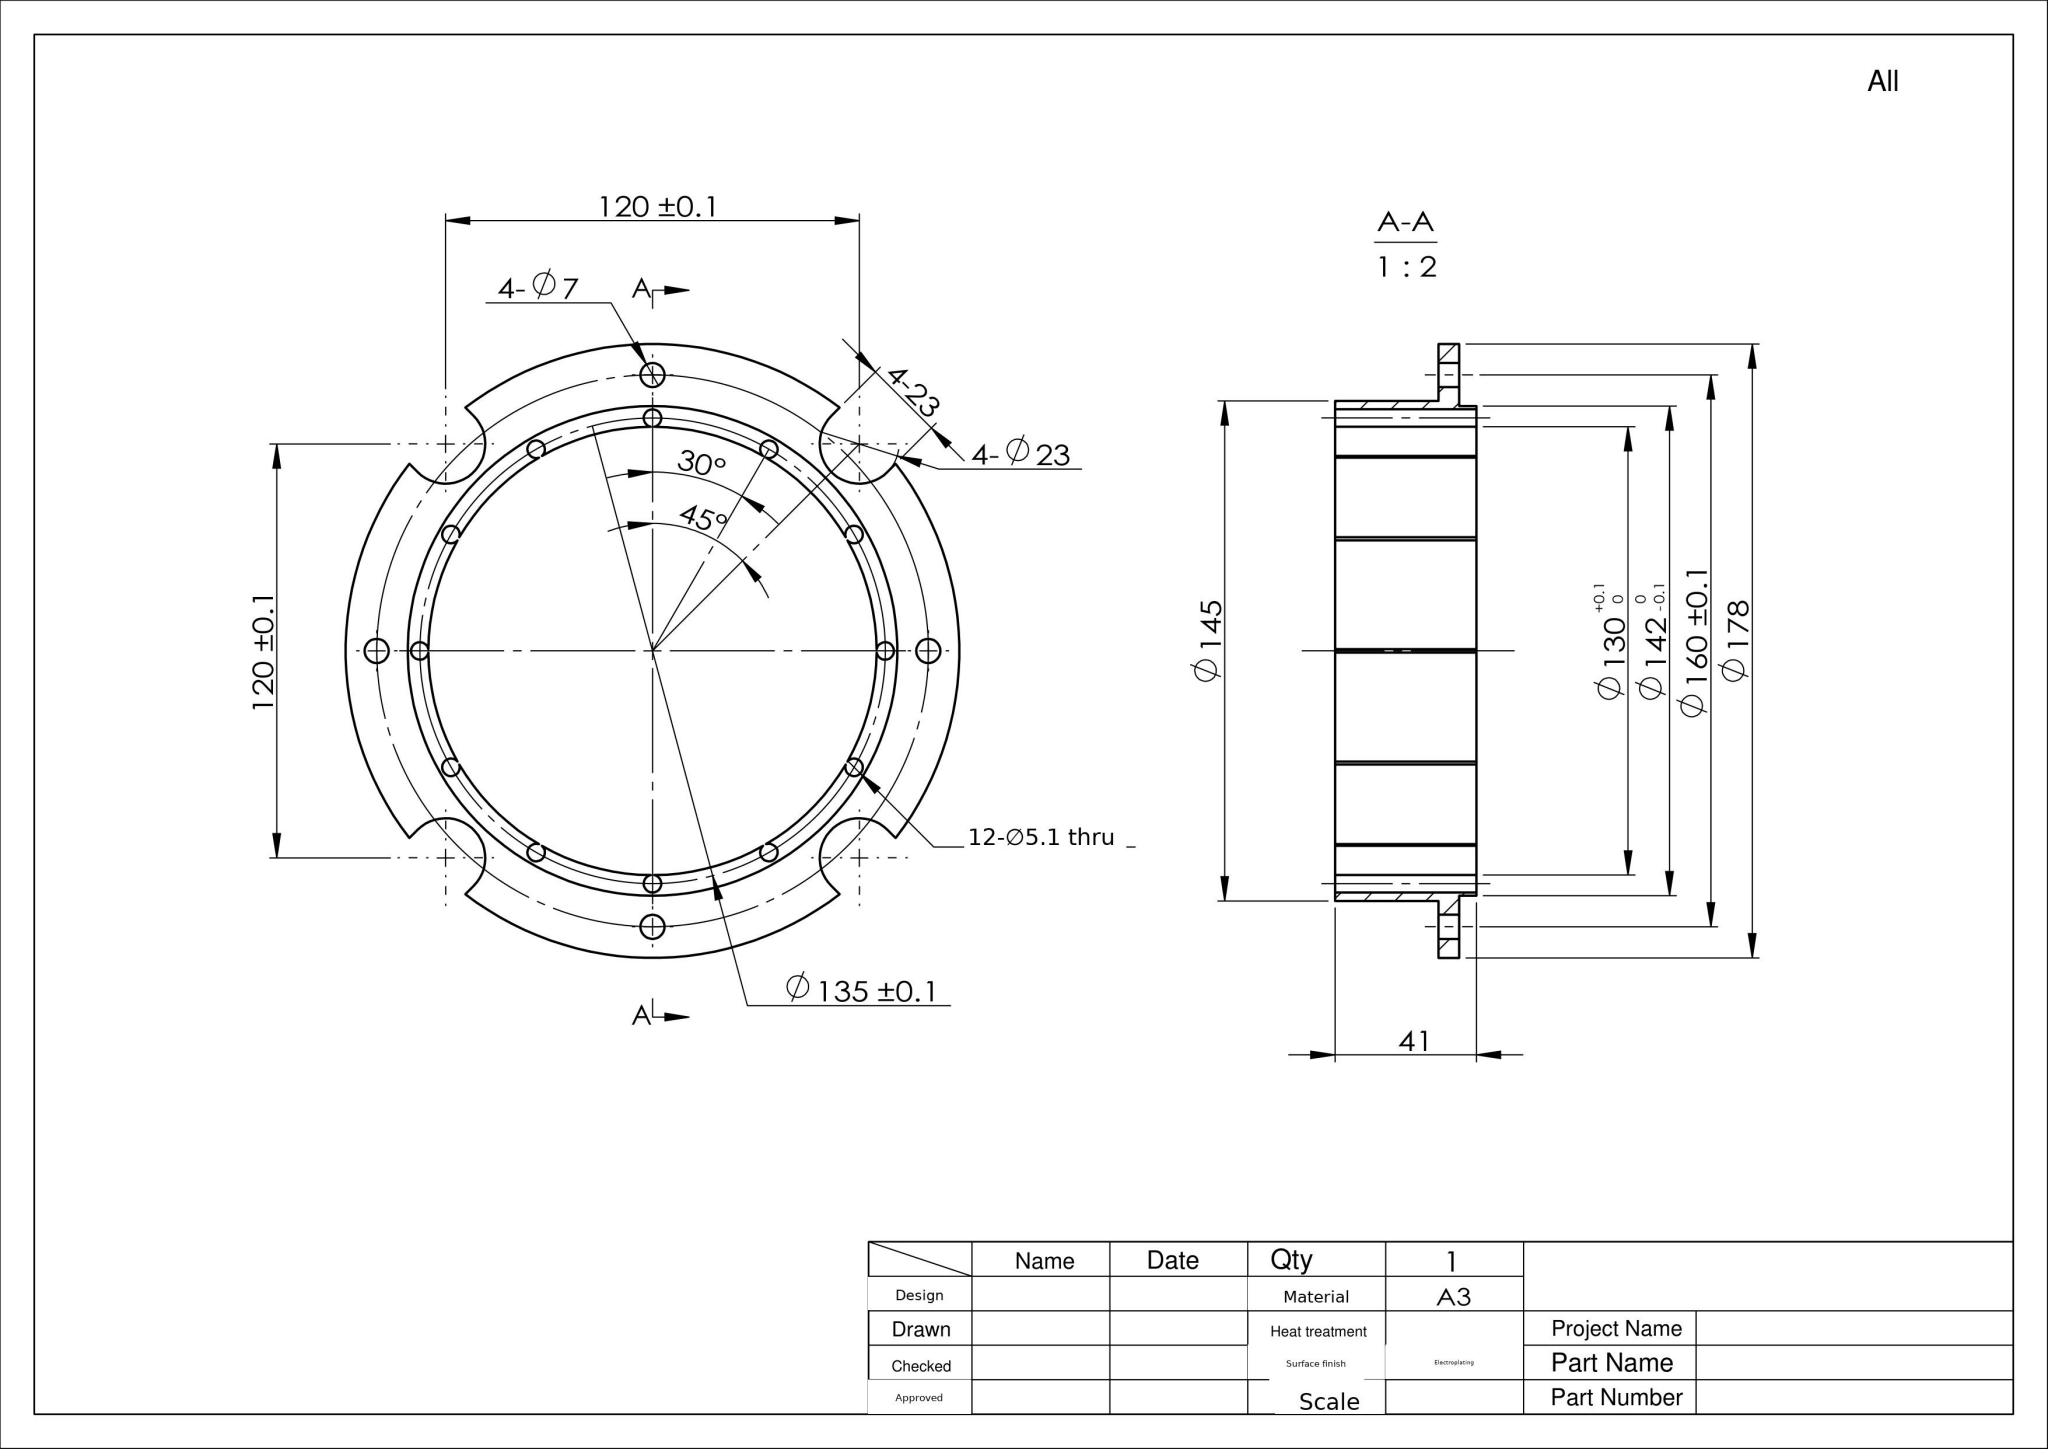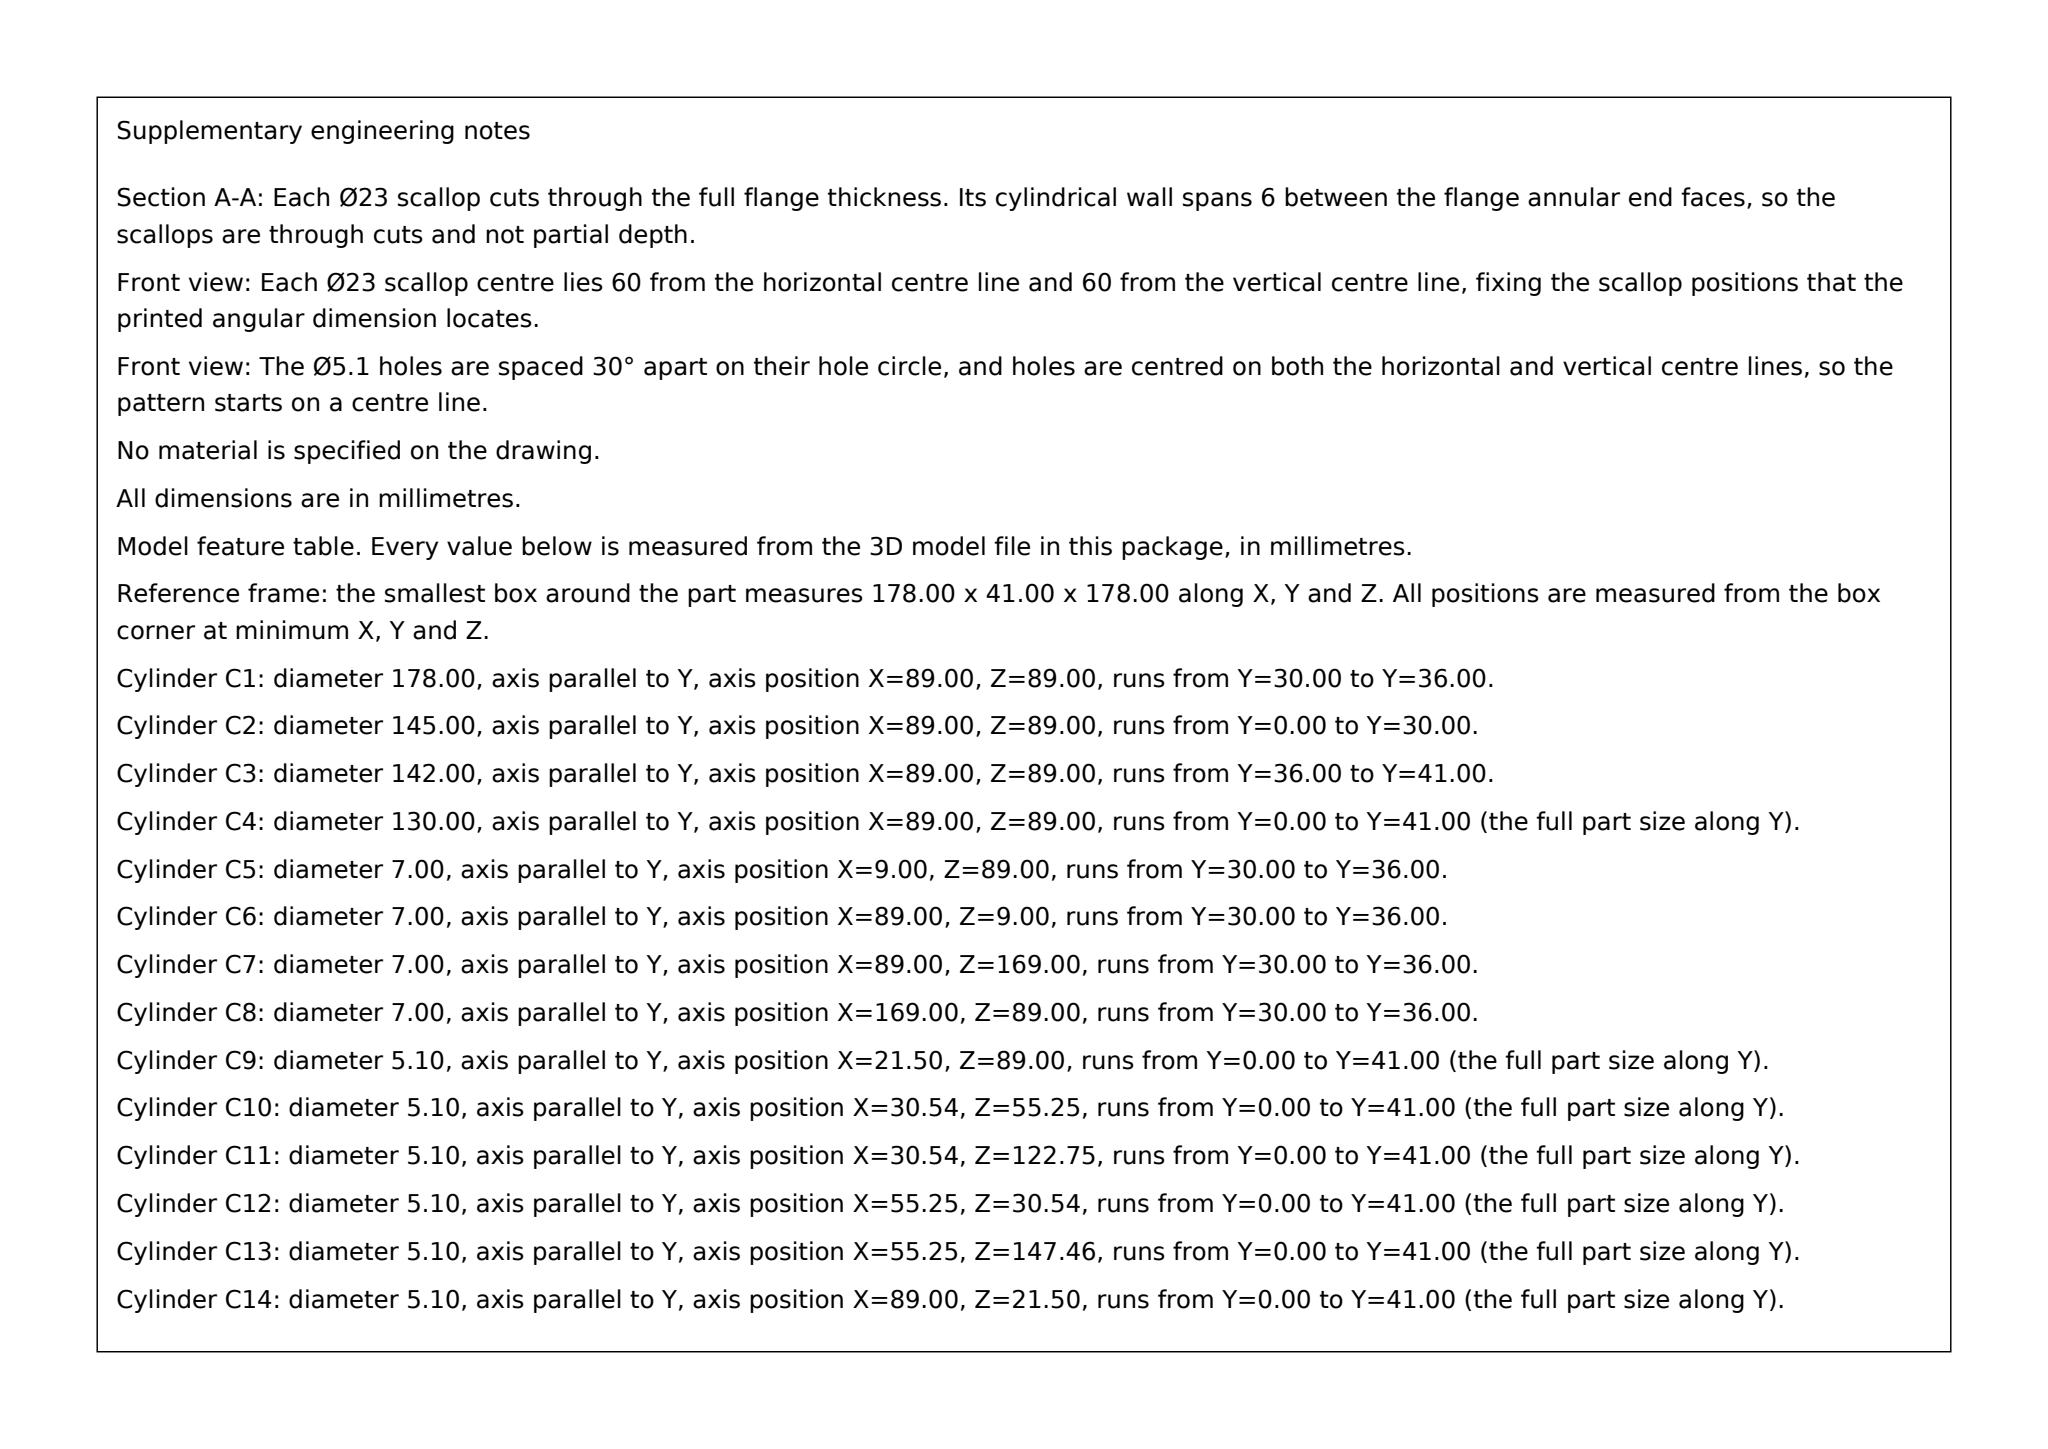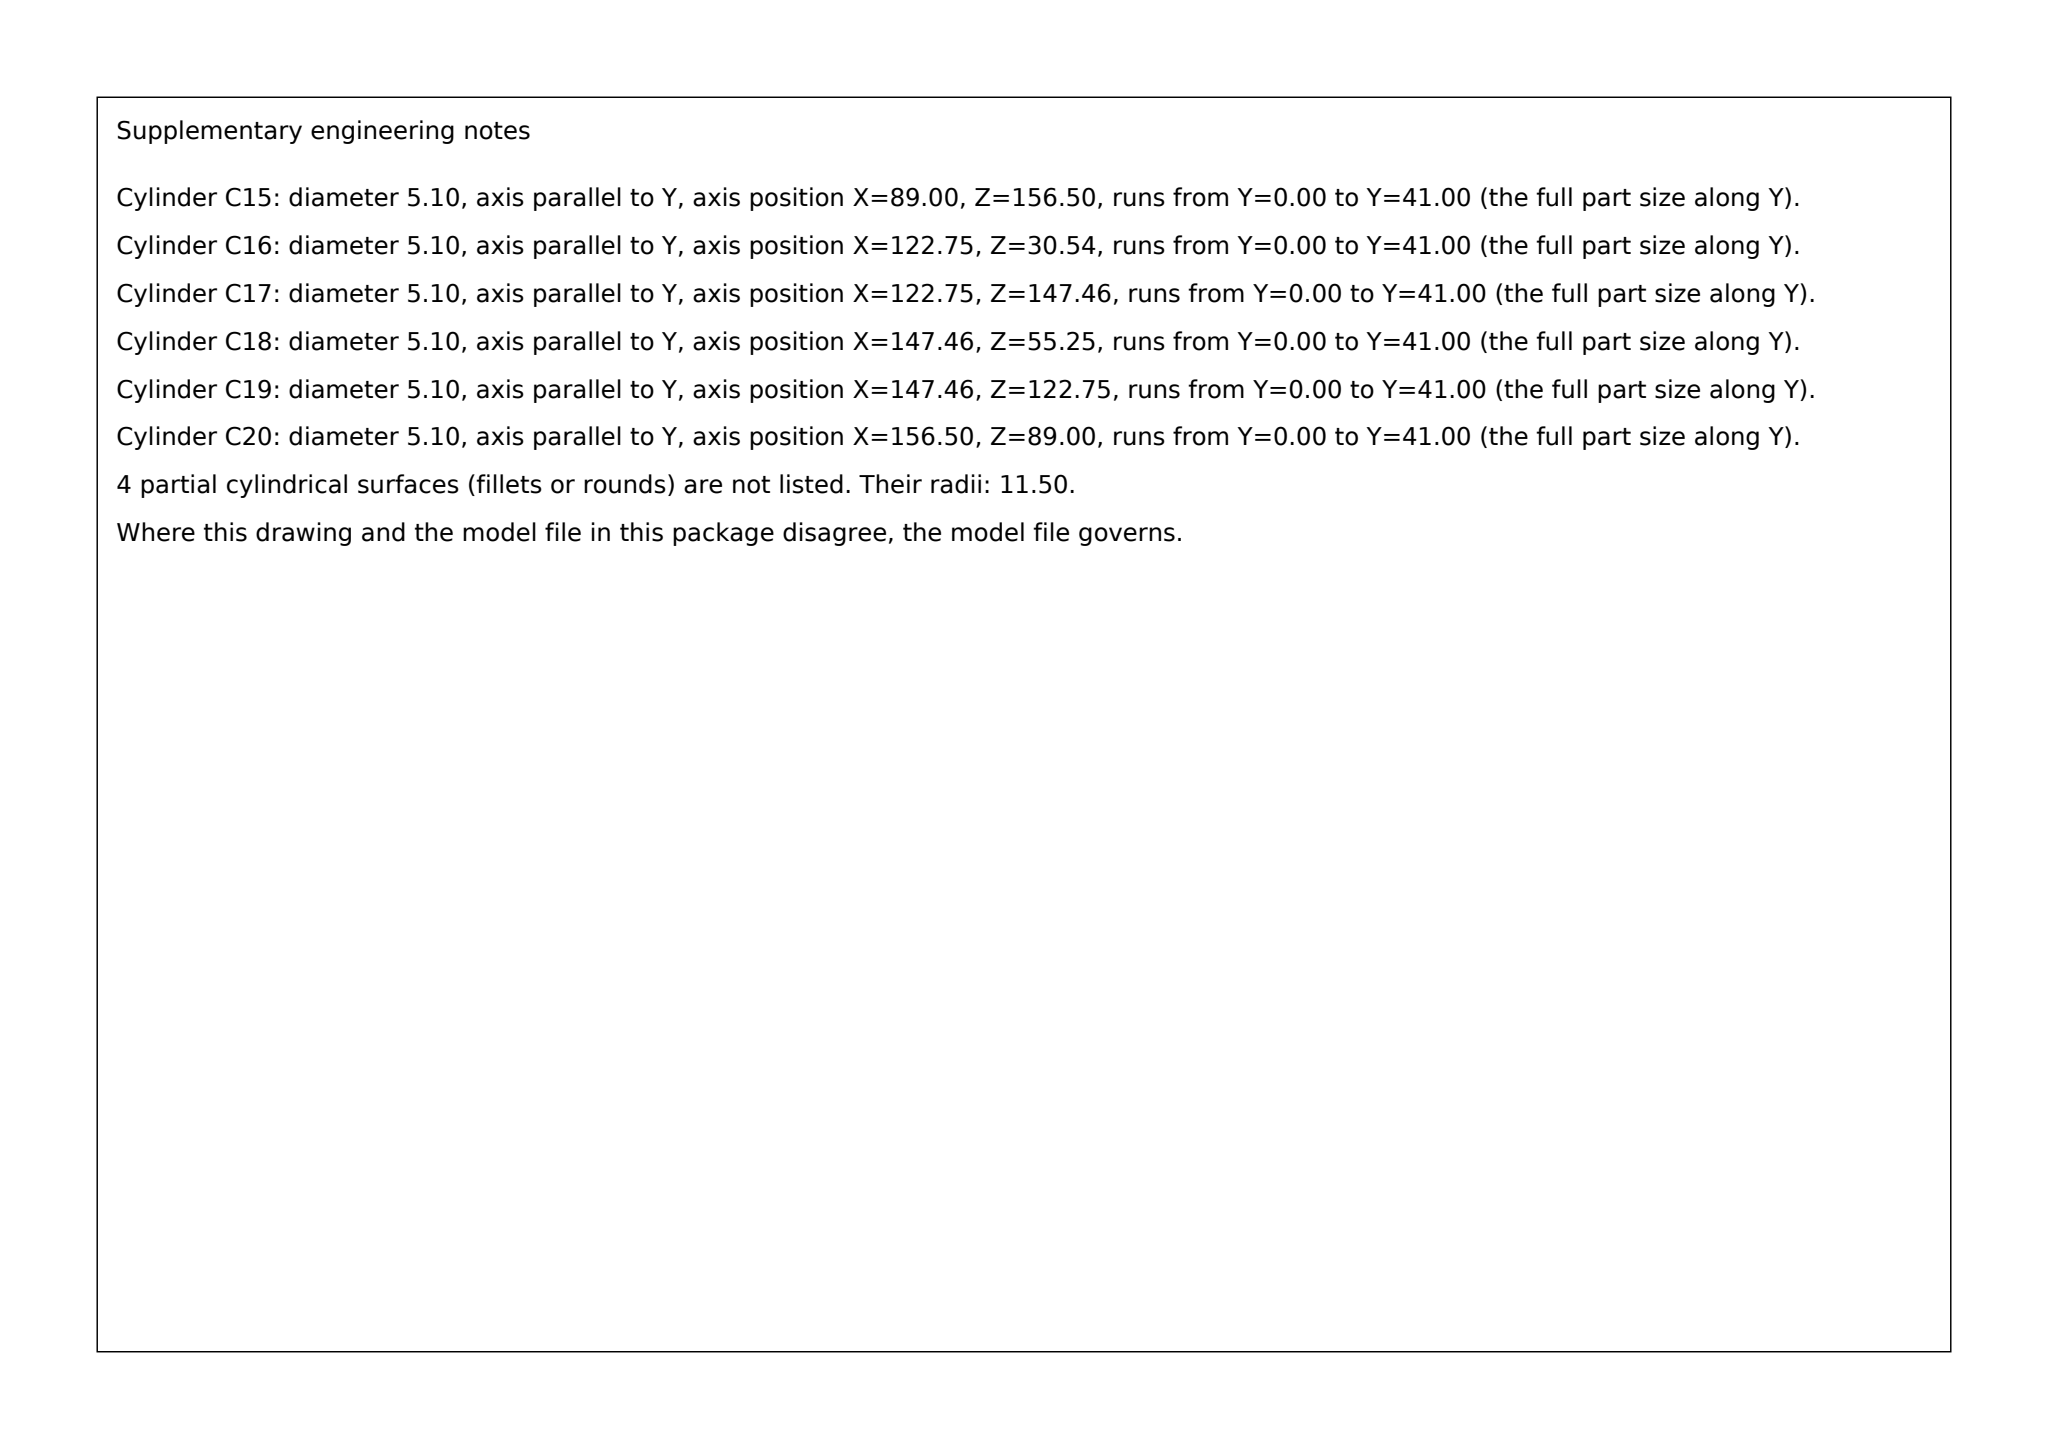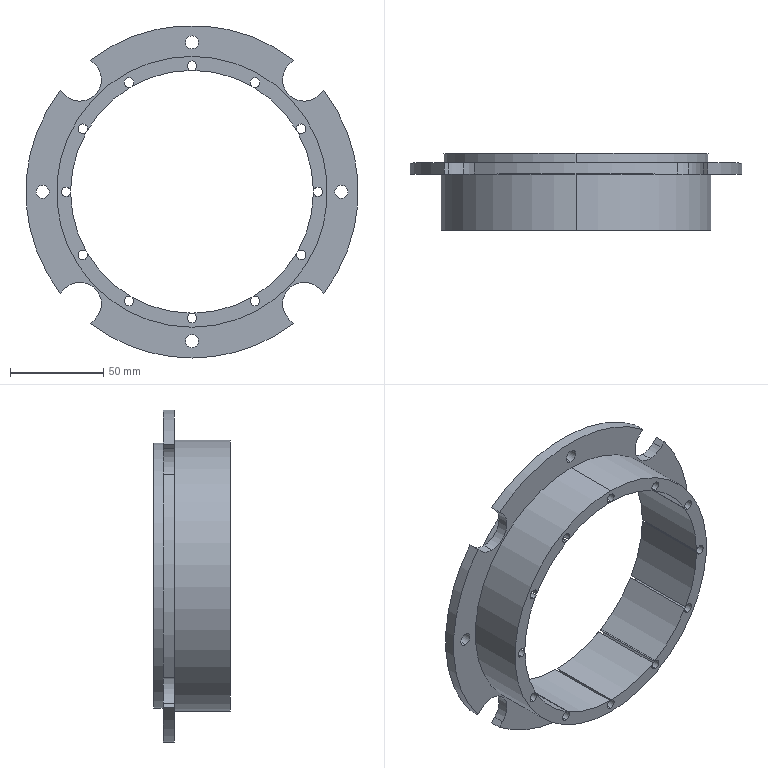Part | SolidWorks | mm | 1 solid | 80 faces | box 178 x 41 x 178 mm | volume 161583 mm3 | cylinder 68 | plane 12 | commonest cylinder face diameters 5.1 x33 130 x12 7 x8 23 x6 178 x5 142 x2 145 x2
Drawing notes:
Ø178 END FLANGES 6 THK EA END, 41 OA | from the solid: cyl dia178 axis y len 6 at each end of 41 bbox; planes y=0,35?,41
Ø145 OD BAND 30 LG; STEP FACES AT 30 & 36 FROM LH END FACE | from the solid: cyl dia145 len 30; axis_planes y=30 and y=36
Ø142 -0.1/0 C'BORE DP 5 EA END OF Ø130 BORE | from the solid: cyl dia142 axis y len 5, 2 off; dia130 len 41 thru
4-Ø7 DP 6 BLIND IN FLANGE | from the solid: cyl dia7 axis y len 6 at (9,89),(89,9),(89,169),(169,89)
4-Ø23 DP 6 BLIND IN FLANGE | from the solid: cyl dia23 axis y len 6 at (29,29),(29,149),(149,29),(149,149)
build123d program:
from build123d import *

# Parameters (mm, degrees)
SKETCH2_R          = 2.55
CUT_EXTRUDE1_DEPTH = 133.374
SKETCH3_R          = 3.5
CUT_EXTRUDE2_DEPTH = 130.391
CUT_EXTRUDE3_DEPTH = 130.391


with BuildPart() as part:
    # Sketch1 → Revolve1 (revolve)
    with BuildSketch(Plane.XY, mode=Mode.PRIVATE) as revolve1_sk:
        Polygon((89, 30), (89, 36), (71, 36), (71, 41), (65, 41), (65, 0), (72.5, 0), (72.5, 30), align=None)
    revolve(revolve1_sk.sketch.rotate(Axis((0, 0, 0), (0, 1, 0)), 90), axis=Axis((0, 0, 0), (0, 1, 0)))

    # Sketch2 → Cut-Extrude1 (cut, through all)
    with BuildSketch(Plane.XZ):
        with Locations((0, 67.5)):
            Circle(SKETCH2_R)
        with Locations((33.75, 58.457)):
            Circle(SKETCH2_R)
        with Locations((58.457, 33.75)):
            Circle(SKETCH2_R)
        with Locations((67.5, 0)):
            Circle(SKETCH2_R)
        with Locations((58.457, -33.75)):
            Circle(SKETCH2_R)
        with Locations((33.75, -58.457)):
            Circle(SKETCH2_R)
        with Locations((0, -67.5)):
            Circle(SKETCH2_R)
        with Locations((-33.75, -58.457)):
            Circle(SKETCH2_R)
        with Locations((-58.457, -33.75)):
            Circle(SKETCH2_R)
        with Locations((-67.5, 0)):
            Circle(SKETCH2_R)
        with Locations((-58.457, 33.75)):
            Circle(SKETCH2_R)
        with Locations((-33.75, 58.457)):
            Circle(SKETCH2_R)
    extrude(amount=-CUT_EXTRUDE1_DEPTH, mode=Mode.SUBTRACT)

    # Sketch3 → Cut-Extrude2 (cut, through all)
    with BuildSketch(Plane.XZ.offset(-30)):
        with Locations(Location((0, 80, 0), (0, 0, 270))):
            Circle(SKETCH3_R)
        with Locations(Location((80, 0, 0), (0, 0, 270))):
            Circle(SKETCH3_R)
        with Locations(Location((0, -80, 0), (0, 0, 270))):
            Circle(SKETCH3_R)
        with Locations(Location((-80, 0, 0), (0, 0, 270))):
            Circle(SKETCH3_R)
    extrude(amount=-CUT_EXTRUDE2_DEPTH, mode=Mode.SUBTRACT)

    # Sketch4 → Cut-Extrude3 (cut, through all)
    with BuildSketch(Plane.XZ.offset(-30)):
        with BuildLine():
            Line((-68.132, 51.868), (-81.804, 65.541))
            Line((-81.804, 65.541), (-65.541, 81.804))
            Line((-65.541, 81.804), (-51.868, 68.132))
            ThreePointArc((-51.868, 68.132), (-51.868, 51.868), (-68.132, 51.868))
        make_face()
        with BuildLine():
            Line((51.868, 68.132), (72.401, 88.665))
            Line((72.401, 88.665), (88.665, 72.401))
            Line((88.665, 72.401), (68.132, 51.868))
            ThreePointArc((68.132, 51.868), (51.868, 51.868), (51.868, 68.132))
        make_face()
        with BuildLine():
            Line((85.877, -69.614), (68.132, -51.868))
            ThreePointArc((68.132, -51.868), (51.868, -51.868), (51.868, -68.132))
            Line((51.868, -68.132), (69.614, -85.877))
            Line((69.614, -85.877), (85.877, -69.614))
        make_face()
        with BuildLine():
            Line((-51.868, -68.132), (-68.051, -84.314))
            Line((-68.051, -84.314), (-84.314, -68.051))
            Line((-84.314, -68.051), (-68.132, -51.868))
            ThreePointArc((-68.132, -51.868), (-51.868, -51.868), (-51.868, -68.132))
        make_face()
    extrude(amount=-CUT_EXTRUDE3_DEPTH, mode=Mode.SUBTRACT)


solid = part.part